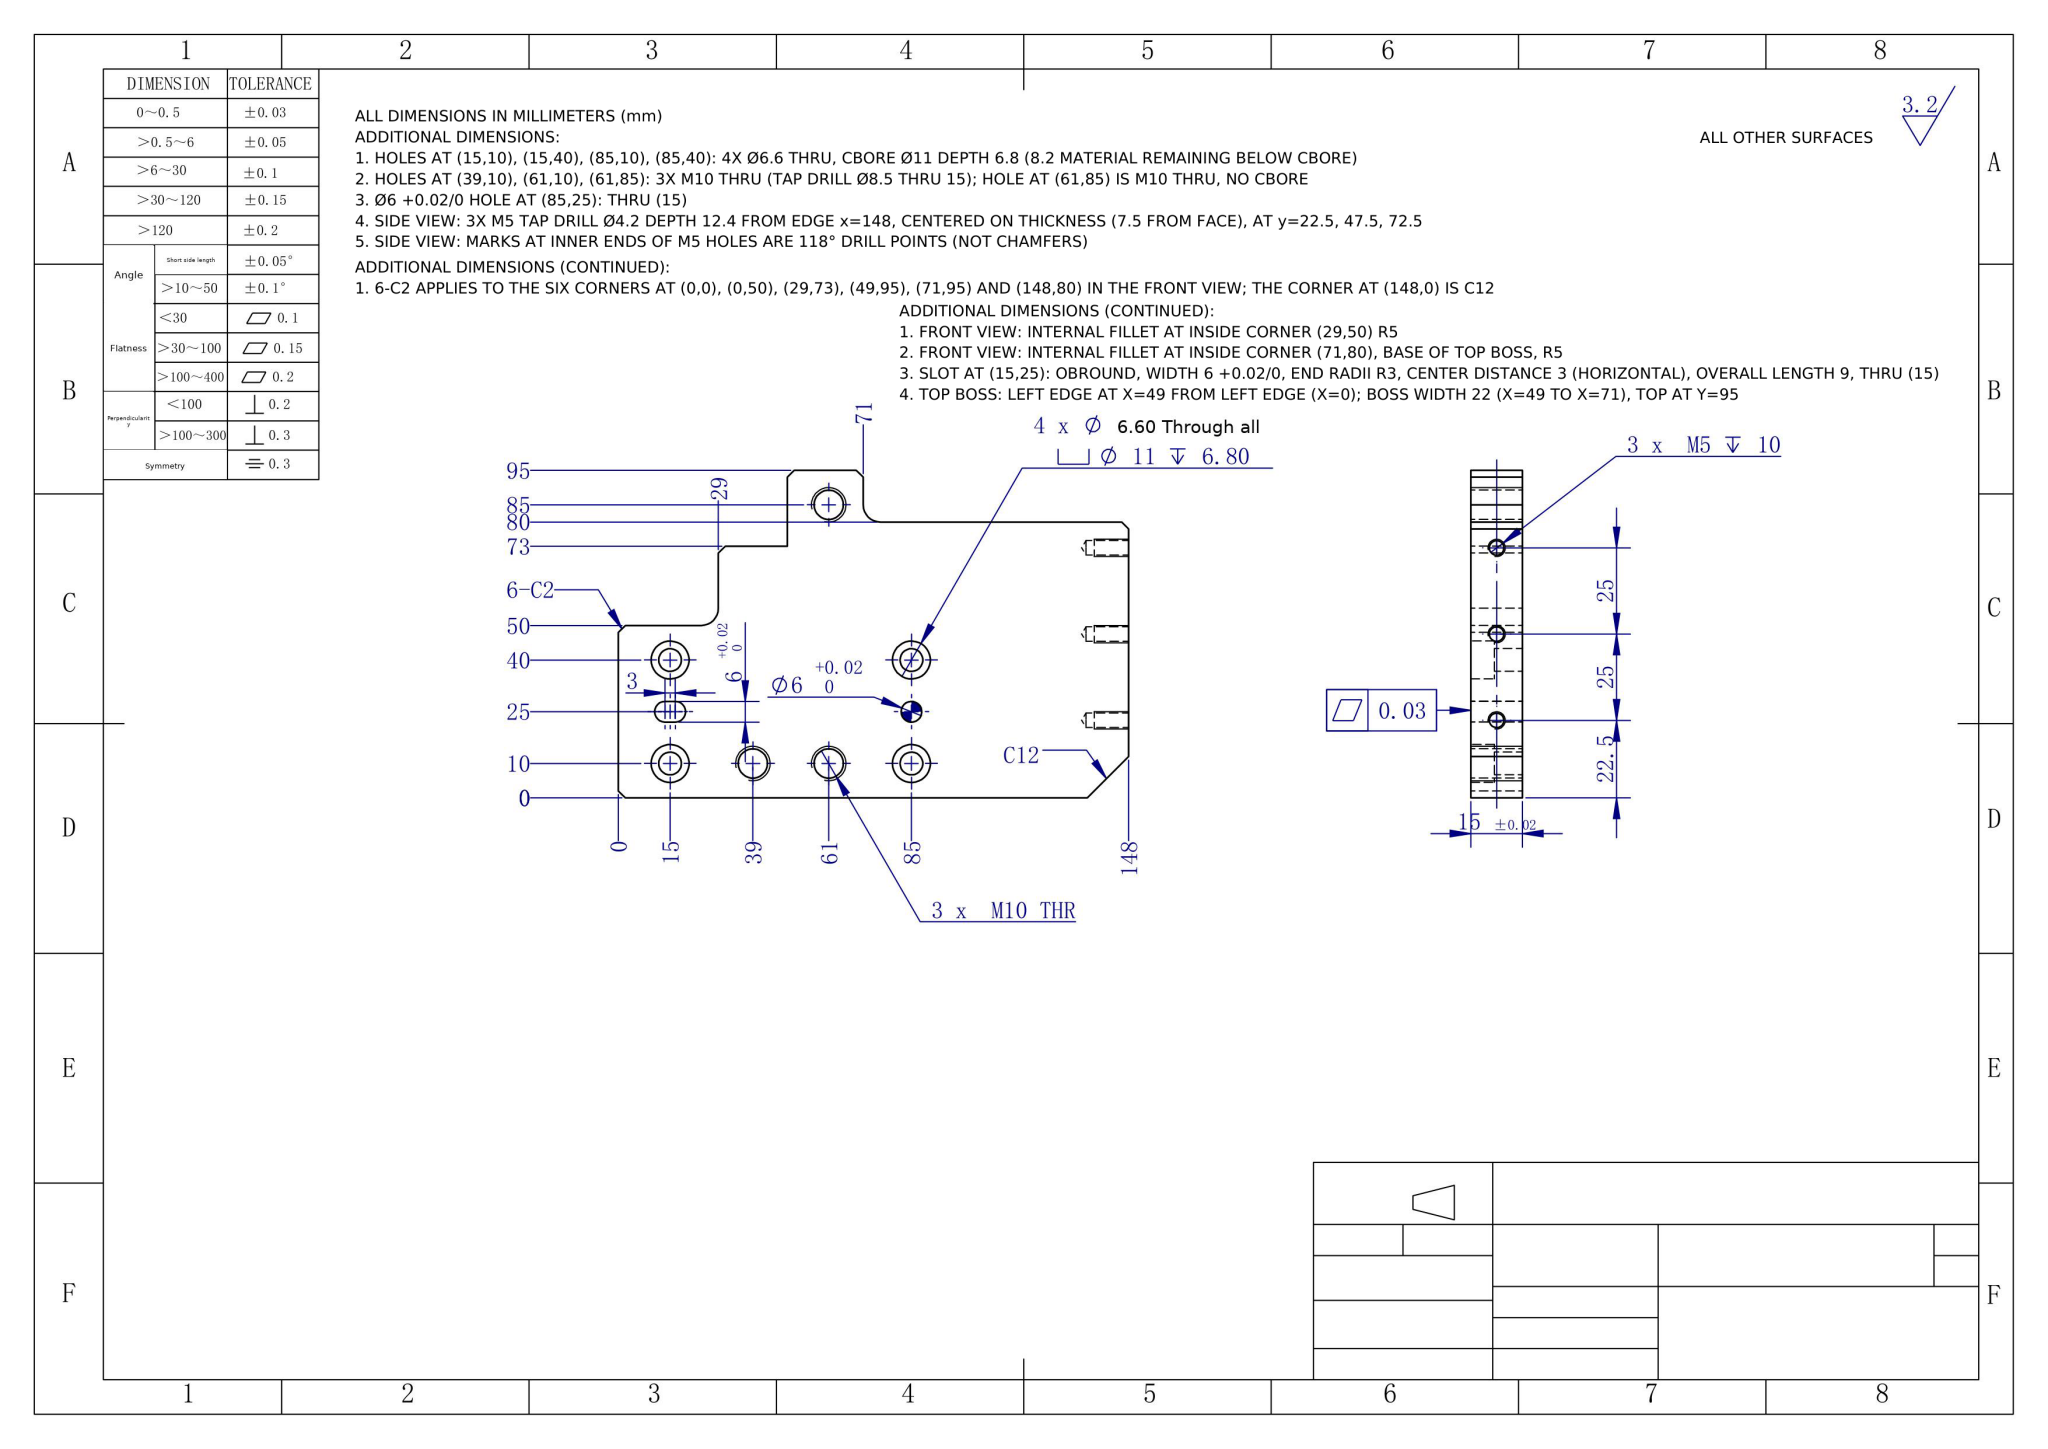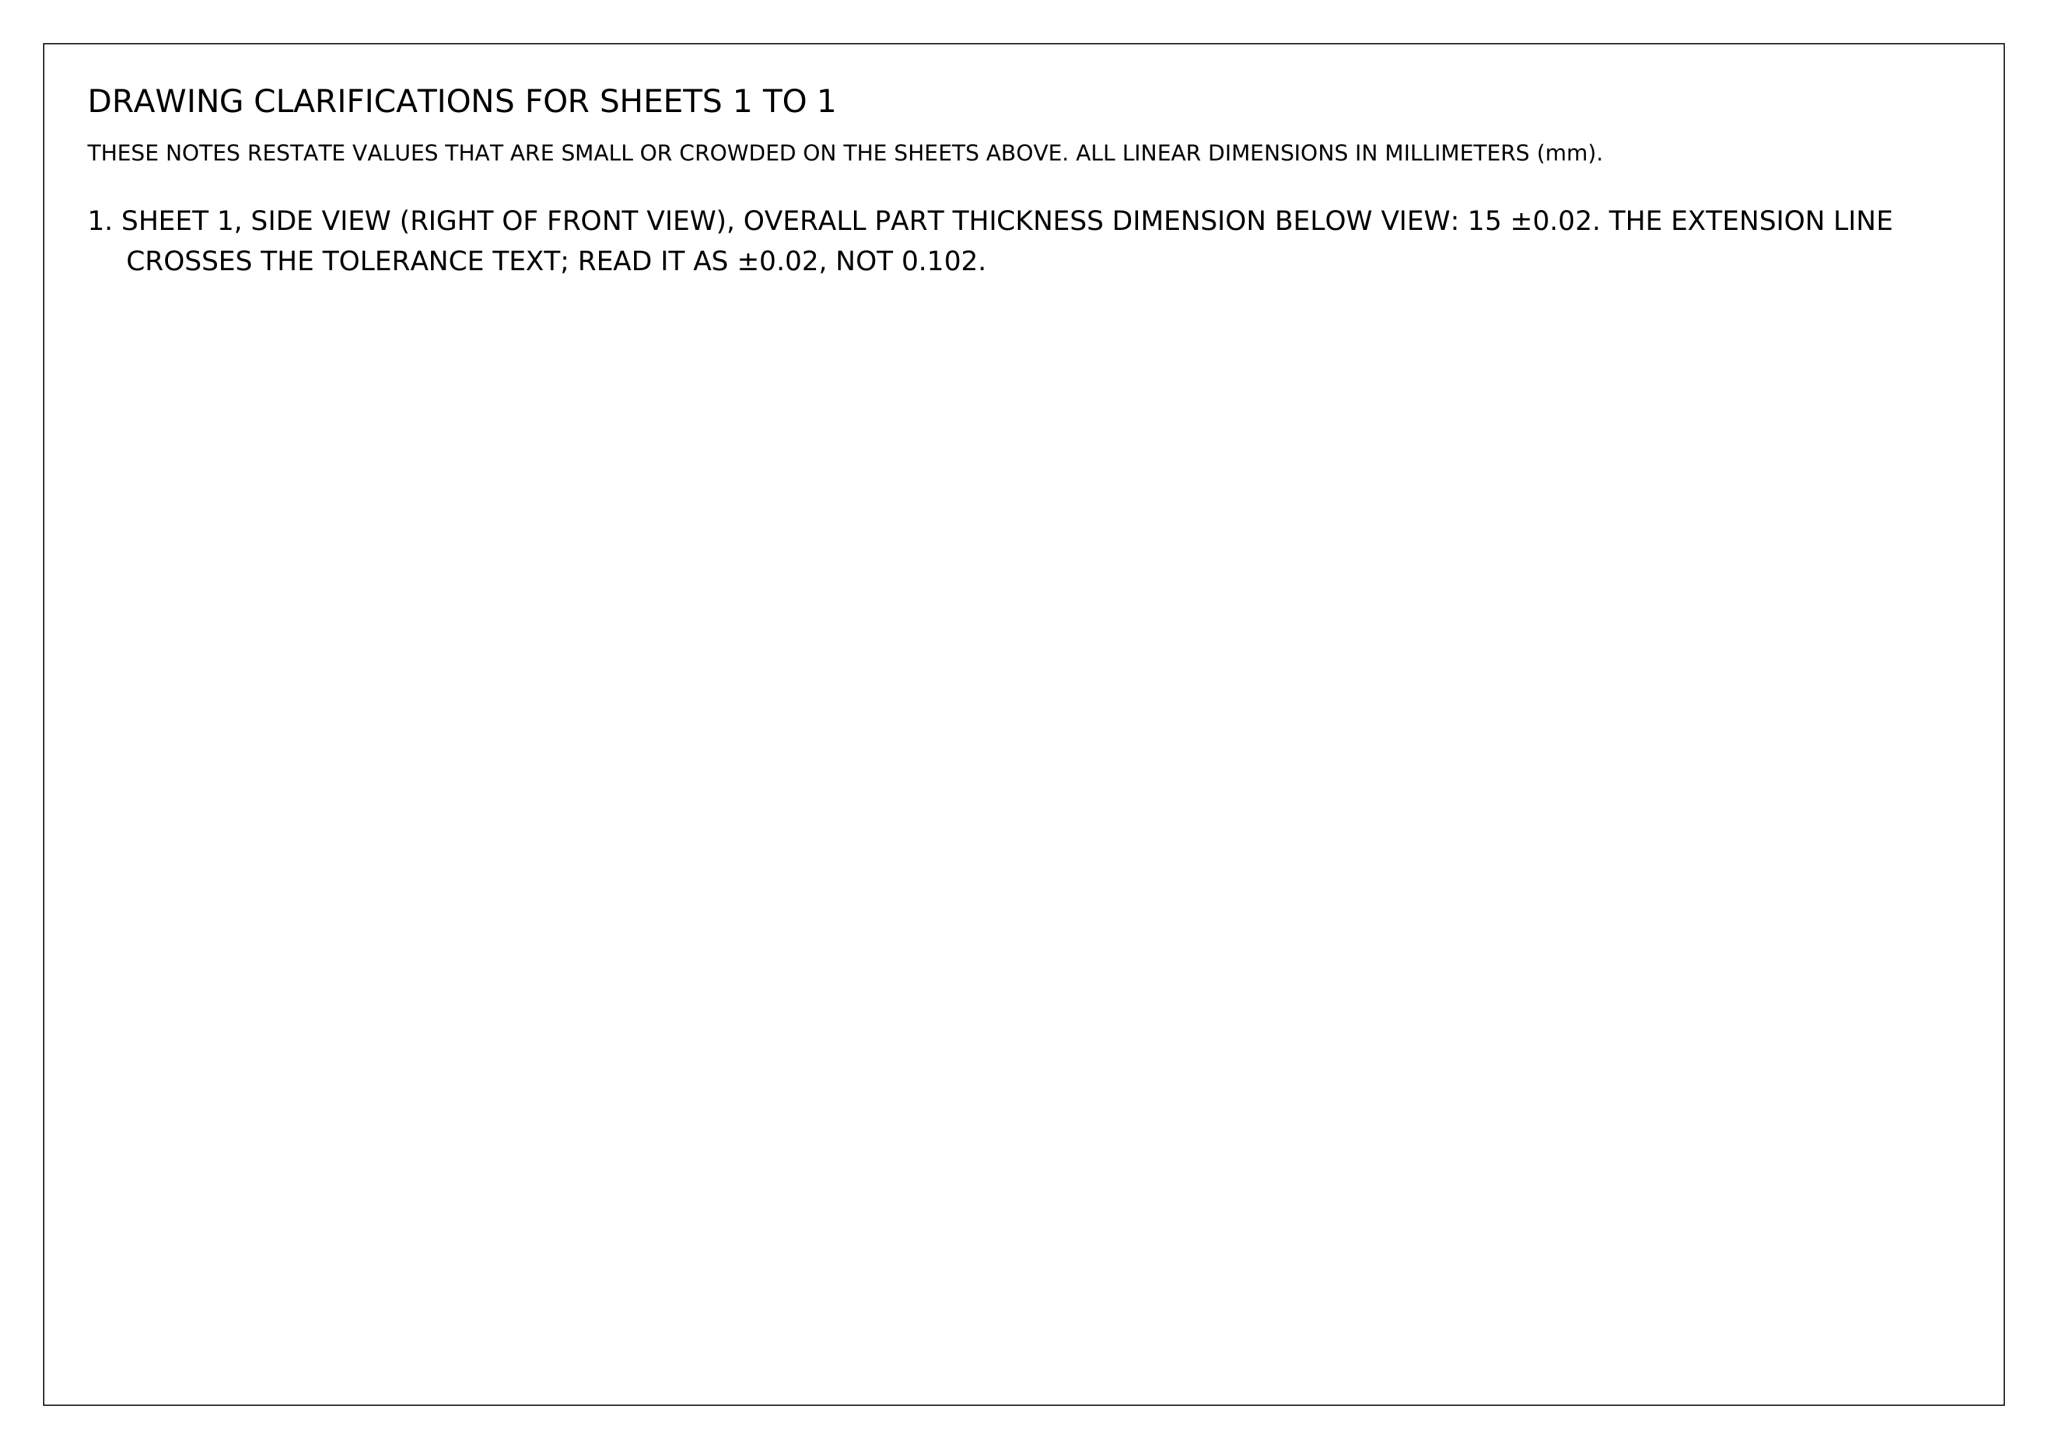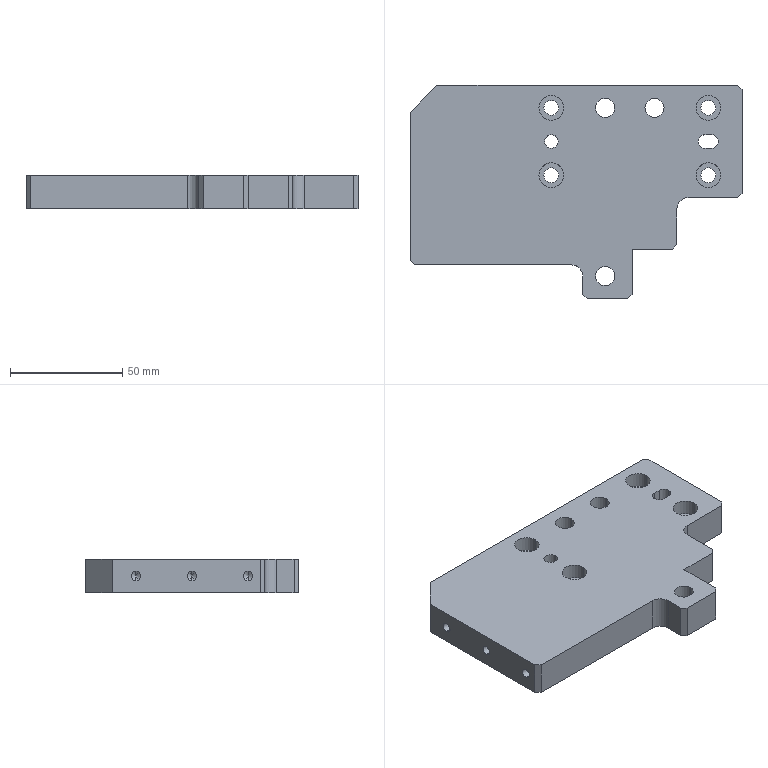Part | NX | mm | 1 solid | 66 faces | box 148 x 95 x 15 mm | volume 158389 mm3 | cylinder 35 | plane 25 | cone 6 | commonest cylinder face diameters 11 x8 6.6 x8 4.2 x6 8.5 x6 6 x5 10 x2